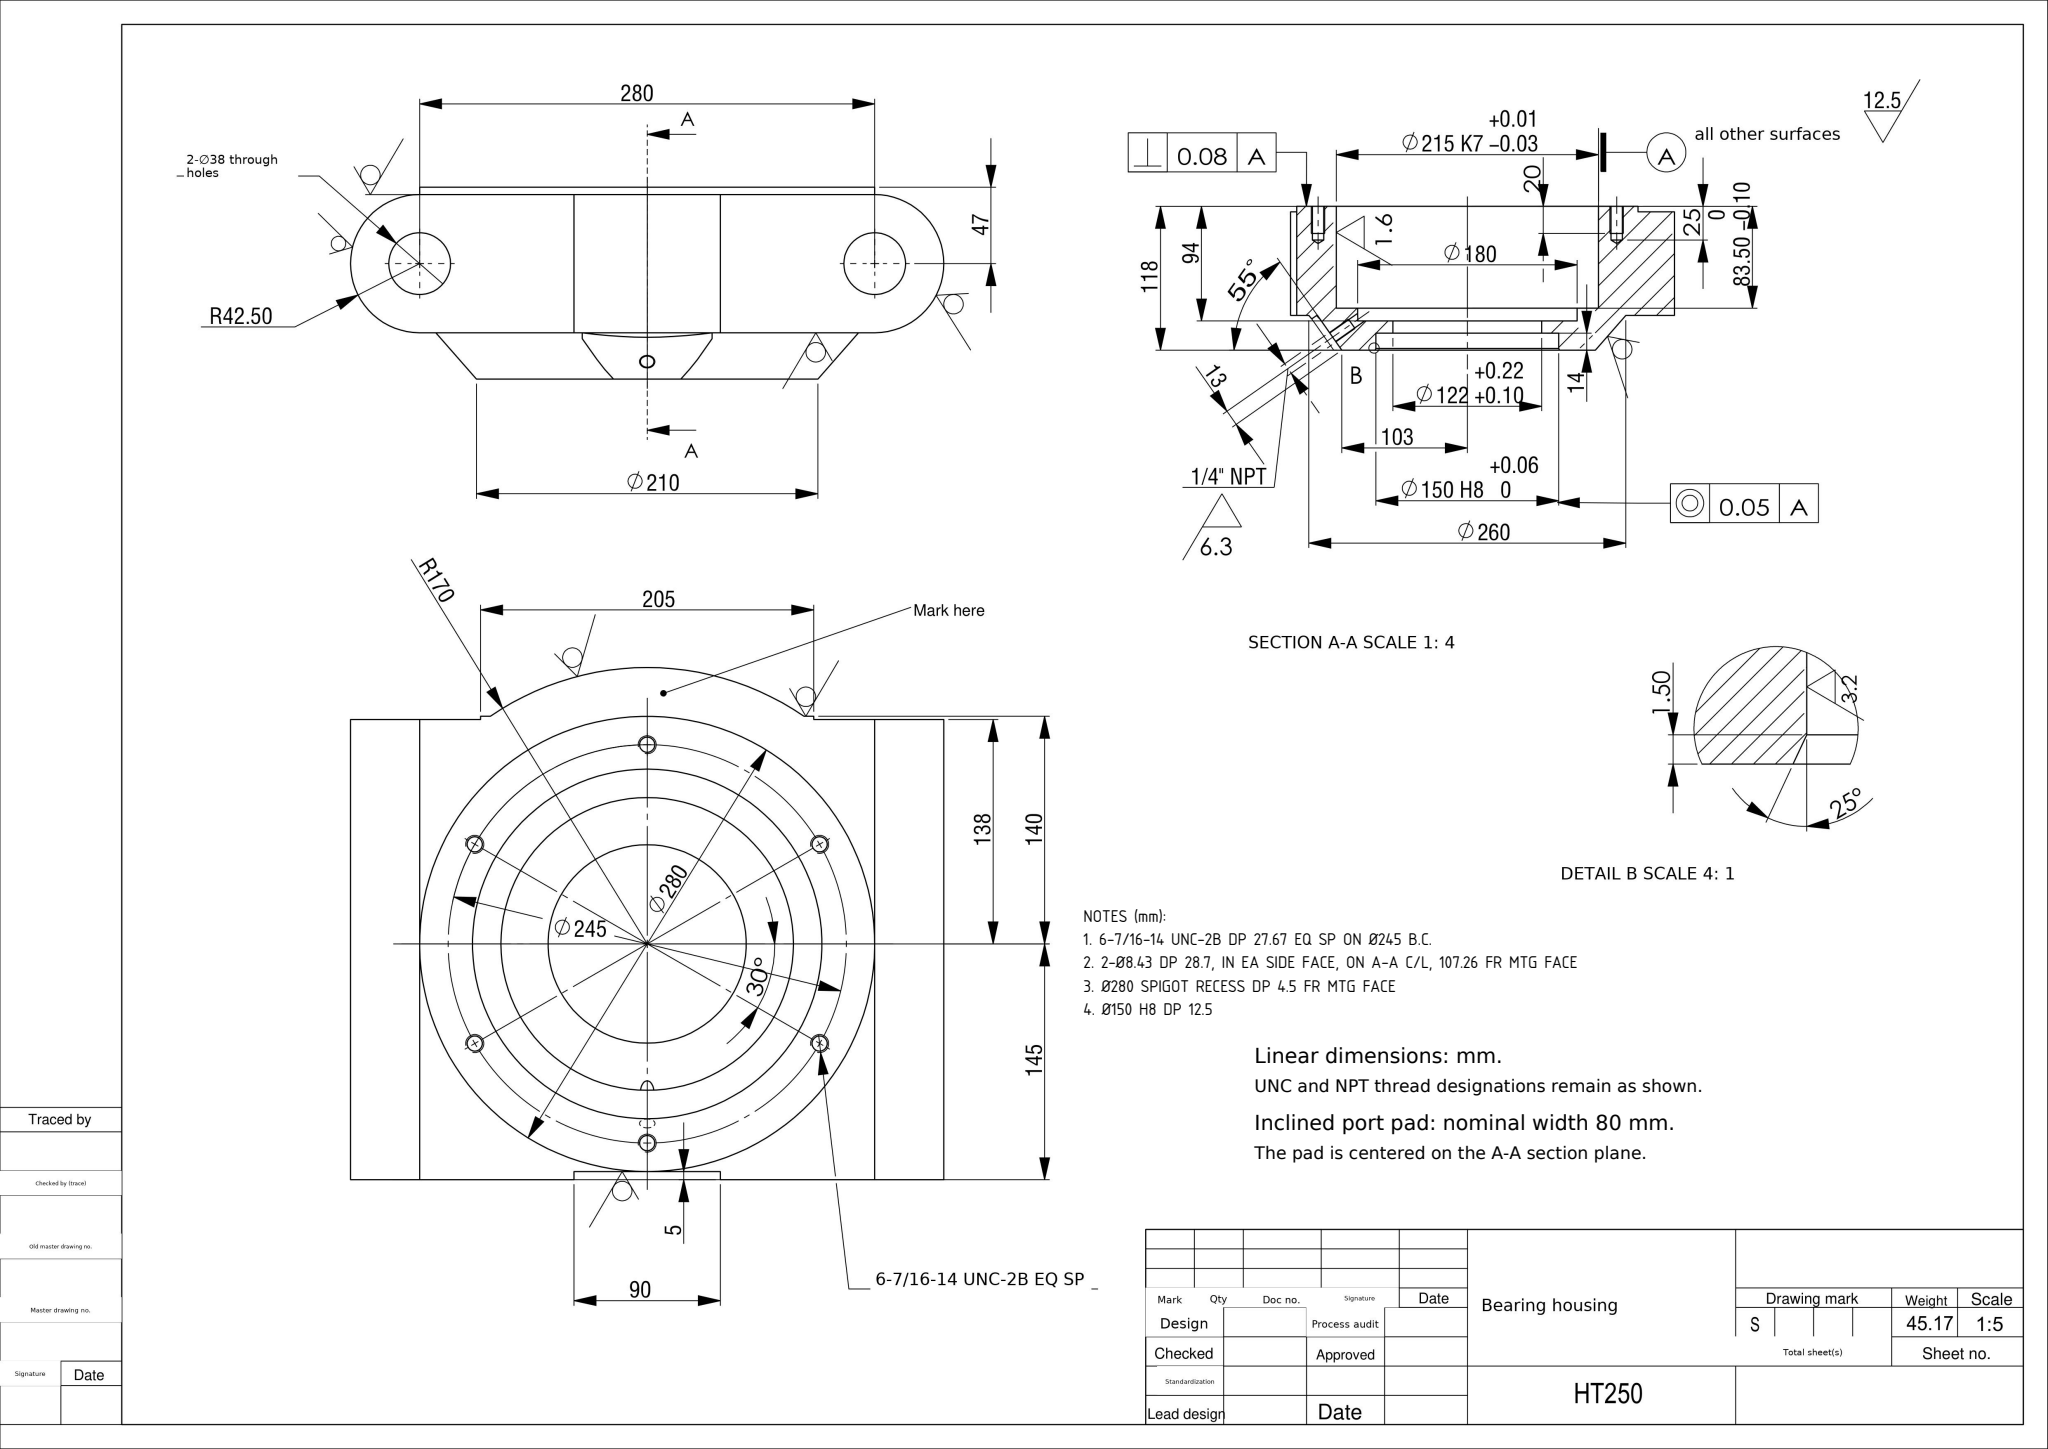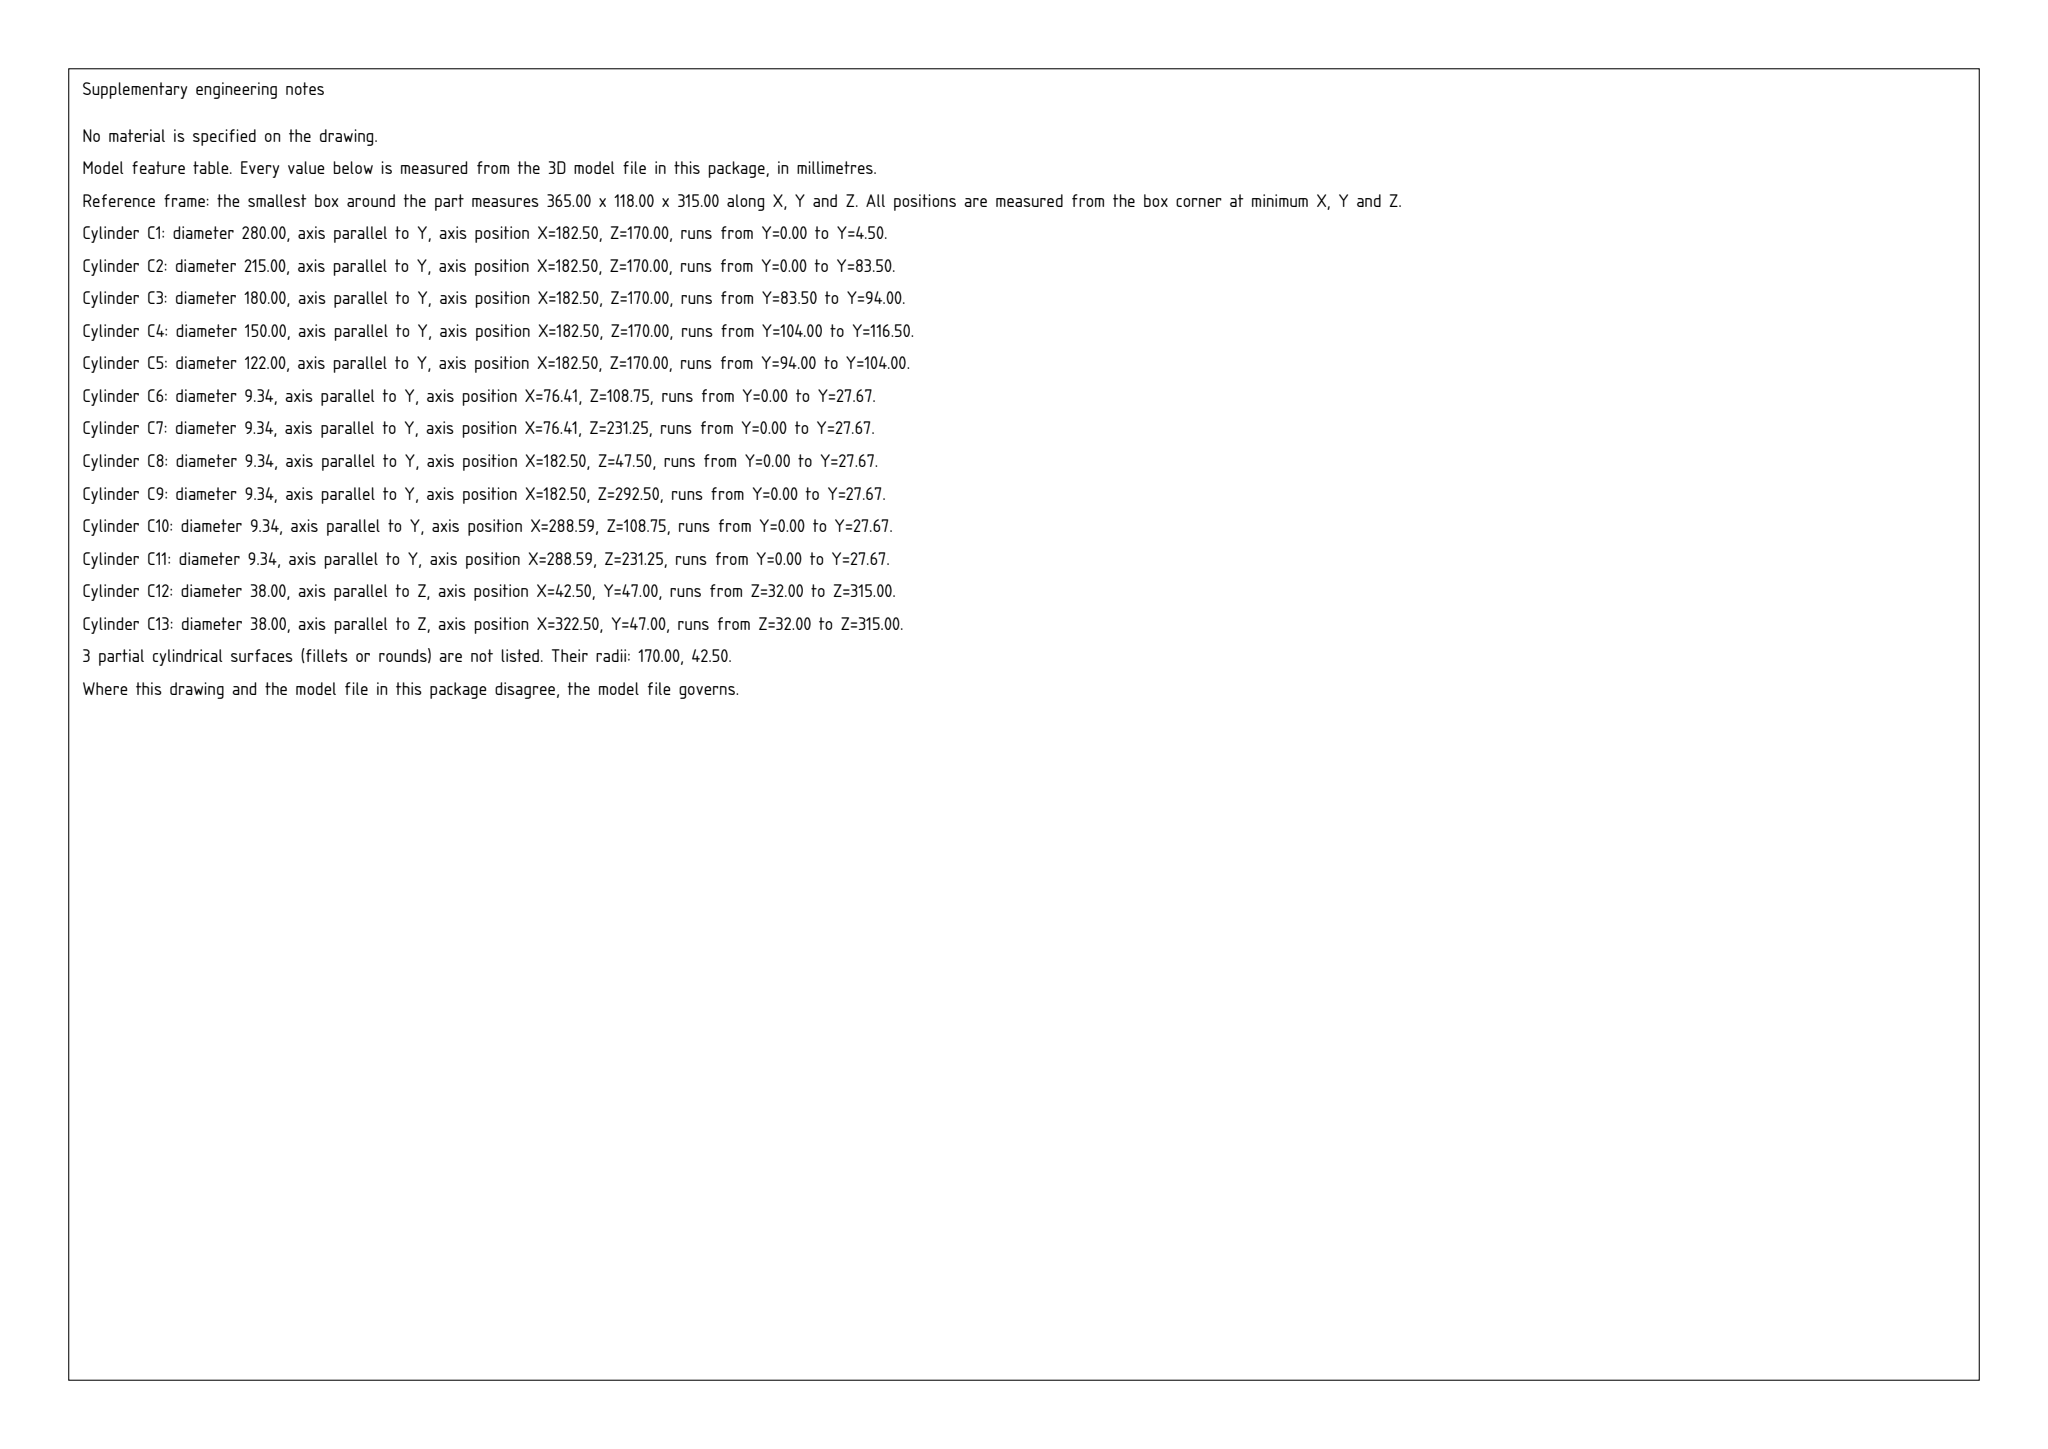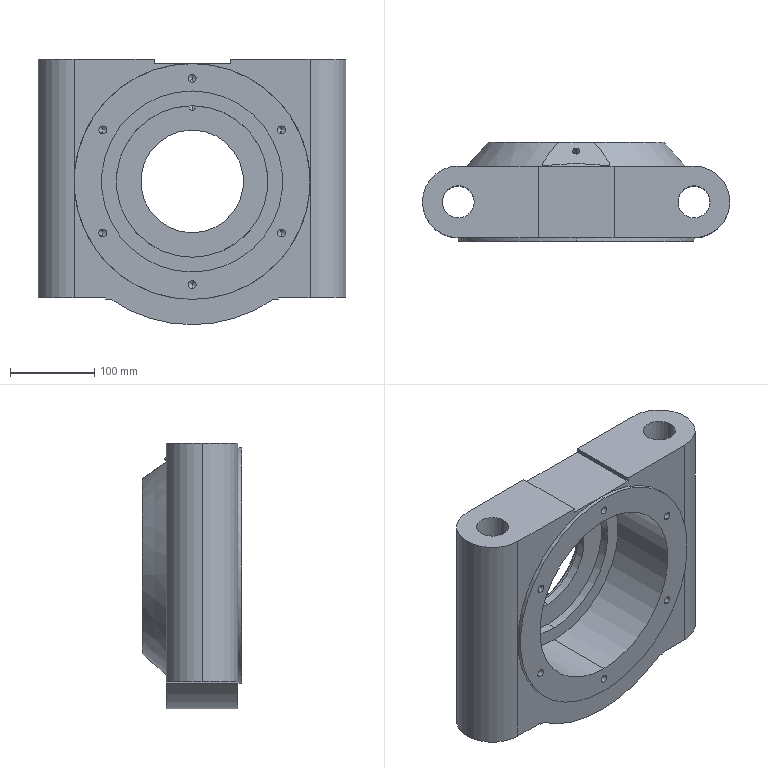Part | SolidWorks | mm | 1 solid | 74 faces | box 365 x 118 x 315 mm | volume 5865953 mm3 | cylinder 33 | plane 24 | cone 17 | commonest cylinder face diameters 9.347 x12 38 x4 85 x3 8.433 x2 340 x2 150 x2 215 x2 280 x2
Drawing notes:
6-7/16-14 UNC-2B DP 27.67 EQ SP ON Ø245 B.C. | from the solid: 6 x cyl dia 9.347 (7/16-14 tap dia), axis y, len 27.67, on R122.5 B.C. about (182.5,170); 118° drill cones
2-Ø8.43 DP 28.7, IN EA SIDE FACE, ON A-A C/L, 107.26 FR MTG FACE | from the solid: cyl dia 8.433, axis z, pos x=182.5 (A-A plane), y=107.26 above y=0 mtg face, len 28.7, count 2
Ø280 SPIGOT RECESS DP 4.5 FR MTG FACE | from the solid: cyl dia 280, axis y, len 4.5, planes y=0 and y=4.5
Ø150 H8 DP 12.5 | from the solid: cyl dia 150, axis y, pos (182.5,170), len 12.5
build123d program:
from build123d import *

# Parameters (mm, degrees)
EXTRUDE1_DEPTH              = 145
EXTRUDE1_DEPTH_BACK         = 140
SKETCH1_R                   = 19
CUT_EXTRUDE2_DEPTH          = 249.105
SKETCH4_W                   = 140
SKETCH4_H                   = 4.5
SKETCH5_5_R                 = 61
CUT_EXTRUDE5_DEPTH          = 262.257
SKETCH5_4_R                 = 90
SKETCH5_4_R_2               = 61
CUT_EXTRUDE7_DEPTH          = 94
SKETCH5_5_2_R               = 107.5
SKETCH5_5_2_R_2             = 90
CUT_EXTRUDE8_DEPTH          = 83.5
CUT_EXTRUDE10_START         = -14
SKETCH11_R                  = 75
SKETCH11_R_2                = 61
CUT_EXTRUDE10_DEPTH         = 14
EXTRUDE2_DEPTH              = 85
CUT_EXTRUDE9_DEPTH          = 2
CIRPATTERN1_COUNT           = 6
CHAMFER1_SIZE               = 1.5
CHAMFER1_SIZE2              = 0.6995
CUT_EXTRUDE13_DEPTH         = 3
CUT_EXTRUDE13_DEPTH_BACK    = 354.868
SKETCH13_W                  = 80
SKETCH13_H                  = 46.857
F_3_8_24_TAPPED_HOLE1_D     = 8.433
F_3_8_24_TAPPED_HOLE1_DEPTH = 50
F_3_8_24_TAPPED_HOLE1_TIP   = 2.533


with BuildPart() as part:
    # Sketch1 → Extrude1 (new, two sides: drawn at the far end of the back side and taken through both)
    with BuildSketch(Plane.XY.offset(-EXTRUDE1_DEPTH_BACK)):
        with BuildLine():
            Line((-140, 42.5), (140, 42.5))
            ThreePointArc((140, 42.5), (182.5, 0), (140, -42.5))
            Line((140, -42.5), (-140, -42.5))
            ThreePointArc((-140, -42.5), (-182.5, 0), (-140, 42.5))
        make_face()
        with Locations((-140, 0)):
            Circle(SKETCH1_R, mode=Mode.SUBTRACT)
        with Locations(Location((140, 0, 0), (0, 0, 180))):
            Circle(SKETCH1_R, mode=Mode.SUBTRACT)
    extrude(amount=EXTRUDE1_DEPTH + EXTRUDE1_DEPTH_BACK)

    # Sketch2 → Cut-Extrude2 (cut, through all)
    with BuildSketch(Plane.XZ.offset(42.5)):
        Polygon((0, 145), (45, 145), (45, 140), (-45, 140), (-45, 145), align=None)
    extrude(amount=-CUT_EXTRUDE2_DEPTH, mode=Mode.SUBTRACT)

    # Sketch4 → Revolve1 (revolve)
    with BuildSketch(Plane(origin=(0, 0, 0), x_dir=(0, 0, -1), z_dir=(1, 0, 0)), mode=Mode.PRIVATE) as revolve1_sk:
        Polygon((0, 71), (105, 71), (130, 42.5), (0, 42.5), align=None)
        with Locations((70, -44.75)):
            Rectangle(SKETCH4_W, SKETCH4_H)
    revolve(revolve1_sk.sketch.rotate(Axis((0, 93.923, 0), (0, -1, 0)), 90), axis=Axis((0, 93.923, 0), (0, -1, 0)))

    # Sketch5_5 → Cut-Extrude5 (cut, through all)
    with BuildSketch(Plane.XZ.offset(47)):
        with Locations(Location((0, 0, 0), (0, 0, 270))):
            Circle(SKETCH5_5_R)
    extrude(amount=-CUT_EXTRUDE5_DEPTH, mode=Mode.SUBTRACT)

    # Sketch5_4 → Cut-Extrude7 (cut)
    with BuildSketch(Plane.XZ.offset(47)):
        with Locations(Location((0, 0, 0), (0, 0, 270))):
            Circle(SKETCH5_4_R)
        with Locations(Location((0, 0, 0), (0, 0, 270))):
            Circle(SKETCH5_4_R_2, mode=Mode.SUBTRACT)
    extrude(amount=-CUT_EXTRUDE7_DEPTH, mode=Mode.SUBTRACT)

    # Sketch5_5 2 → Cut-Extrude8 (cut)
    with BuildSketch(Plane.XZ.offset(47)):
        with Locations(Location((0, 0, 0), (0, 0, 270))):
            Circle(SKETCH5_5_2_R)
        with Locations(Location((0, 0, 0), (0, 0, 270))):
            Circle(SKETCH5_5_2_R_2, mode=Mode.SUBTRACT)
    extrude(amount=-CUT_EXTRUDE8_DEPTH, mode=Mode.SUBTRACT)

    # Sketch11 → Cut-Extrude10 (cut)
    with BuildSketch(Plane(origin=(0, 71, 0), x_dir=(-1, 0, 0), z_dir=(0, 1, 0)).offset(CUT_EXTRUDE10_START)):
        with Locations(Location((0, 0, 0), (0, 0, 90))):
            Circle(SKETCH11_R)
        with Locations(Location((0, 0, 0), (0, 0, 270))):
            Circle(SKETCH11_R_2, mode=Mode.SUBTRACT)
    extrude(amount=CUT_EXTRUDE10_DEPTH, mode=Mode.SUBTRACT)

    # Sketch6 → Extrude2 (add)
    with BuildSketch(Plane.XZ.offset(42.5)):
        with BuildLine():
            Line((-96.437, -140), (96.437, -140))
            ThreePointArc((96.437, -140), (0, -170), (-96.437, -140))
        make_face()
    extrude(amount=-EXTRUDE2_DEPTH)

    # Sketch7 → Cut-Extrude9 (cut)
    with BuildSketch(Plane(origin=(0, 0, -140), x_dir=(-1, 0, 0), z_dir=(0, 0, -1))):
        with BuildLine():
            Line((140, 42.5), (102.5, 42.5))
            Line((102.5, 42.5), (102.5, -42.5))
            Line((102.5, -42.5), (140, -42.5))
            ThreePointArc((140, -42.5), (182.5, 0), (140, 42.5))
        make_face()
        with BuildLine():
            Line((-102.5, -42.5), (-140, -42.5))
            ThreePointArc((-140, -42.5), (-182.5, 0), (-140, 42.5))
            Line((-140, 42.5), (-102.5, 42.5))
            Line((-102.5, 42.5), (-102.5, -42.5))
        make_face()
    extrude(amount=-CUT_EXTRUDE9_DEPTH, mode=Mode.SUBTRACT)

    # Sketch9 → 7_16-14 Tapped Hole1 (revolve, cut)
    with BuildSketch(Plane(origin=(-106.088, -47, 61.25), x_dir=(0, 0, -1), z_dir=(1, 0, 0))):
        Polygon((0, 0), (0, 30.474), (4.674, 27.666), (4.674, 0), align=None)
    f_7_16_14_tapped_hole1 = revolve(axis=Axis((-106.088, -53.35, 61.25), (0, 1, 0)), mode=Mode.SUBTRACT)

    # CirPattern1: 7_16-14 Tapped Hole1 ×6 about axis
    cirpattern1_axis = Axis((0, 0, 0), (0, 1, 0))
    for i in range(1, CIRPATTERN1_COUNT):
        add(f_7_16_14_tapped_hole1.rotate(cirpattern1_axis, i * 360 / CIRPATTERN1_COUNT), mode=Mode.SUBTRACT)

    # Chamfer1
    chamfer1_edges = [part.edges().sort_by_distance(p)[0] for p in [
        (0, 71, -75),
    ]]
    chamfer1_side = [part.faces().sort_by_distance(p)[0] for p in [
        (0, 64, -75),
    ]]
    chamfer(chamfer1_edges, length=CHAMFER1_SIZE, length2=CHAMFER1_SIZE2, reference=chamfer1_side[0])

    # Sketch13 → Cut-Extrude13 (cut, two sides: drawn at the far end of the back side and taken through both)
    with BuildSketch(Plane(origin=(0, 61.979, 112.913), x_dir=(-1, 0, 0), z_dir=(0, -0.5736, -0.8192)).offset(-CUT_EXTRUDE13_DEPTH_BACK)):
        with Locations((0, 1.289)):
            Rectangle(SKETCH13_W, SKETCH13_H)
    extrude(amount=CUT_EXTRUDE13_DEPTH + CUT_EXTRUDE13_DEPTH_BACK, mode=Mode.SUBTRACT)

    # 3_8-24 Tapped Hole1
    with Locations(Plane(origin=(0, 60.258, 110.456), x_dir=(0, 0.8192, -0.5736), z_dir=(0, 0.5736, 0.8192))):
        with Locations((0, 0)):
            Hole(F_3_8_24_TAPPED_HOLE1_D / 2, depth=F_3_8_24_TAPPED_HOLE1_DEPTH)
            with Locations((0, 0, -(F_3_8_24_TAPPED_HOLE1_DEPTH + F_3_8_24_TAPPED_HOLE1_TIP / 2))):  # 118° drill point
                Cone(0, F_3_8_24_TAPPED_HOLE1_D / 2, F_3_8_24_TAPPED_HOLE1_TIP, mode=Mode.SUBTRACT)


solid = part.part